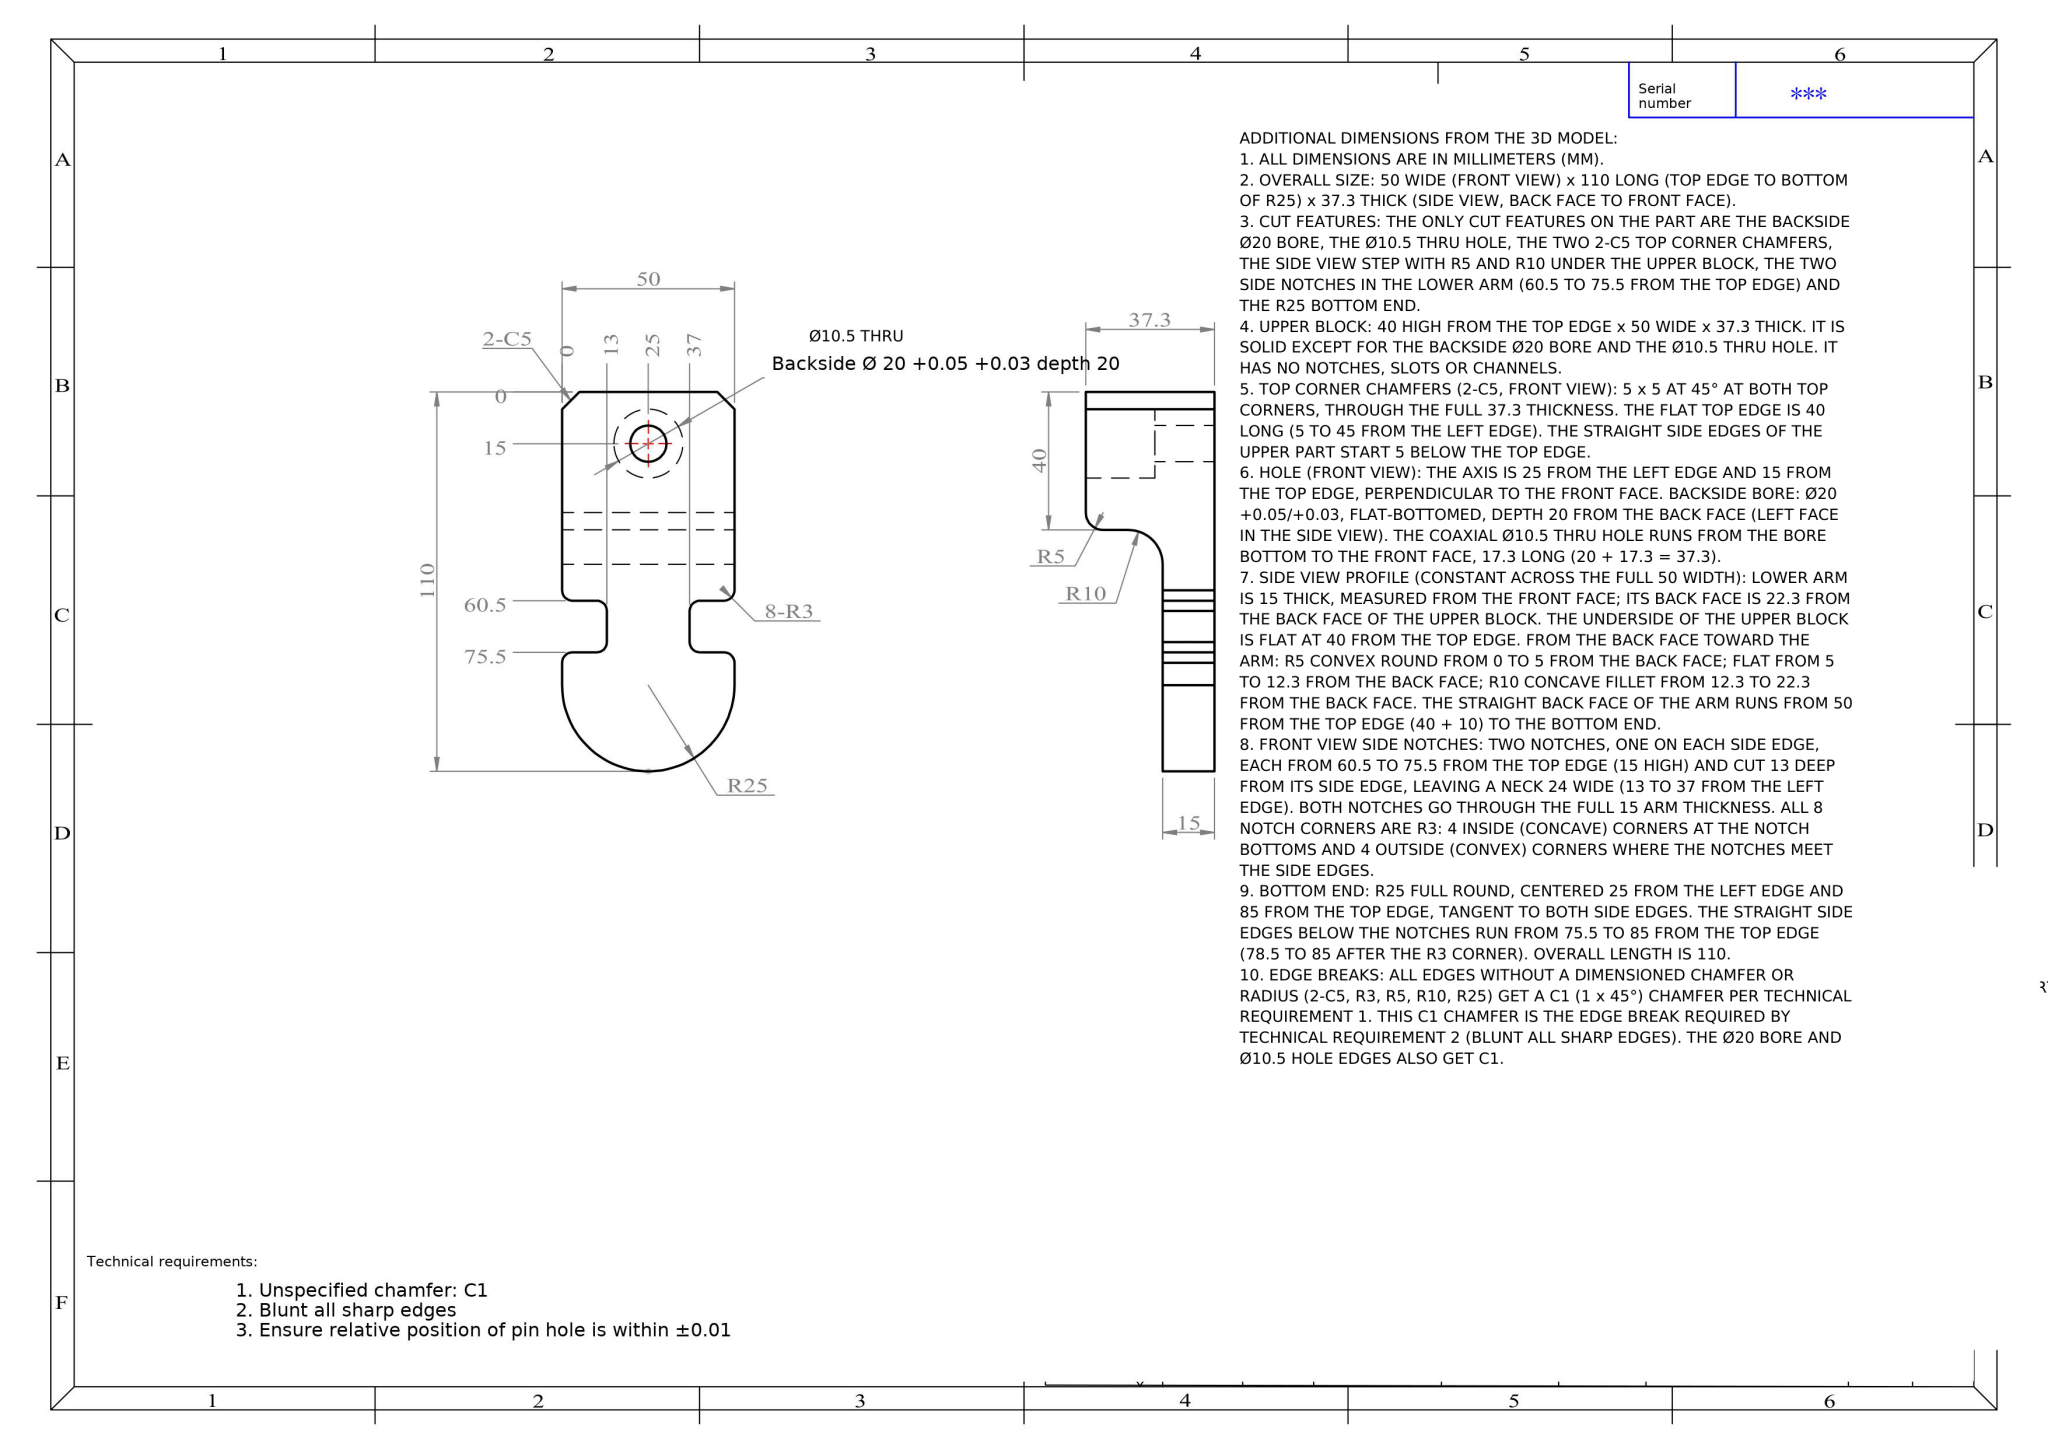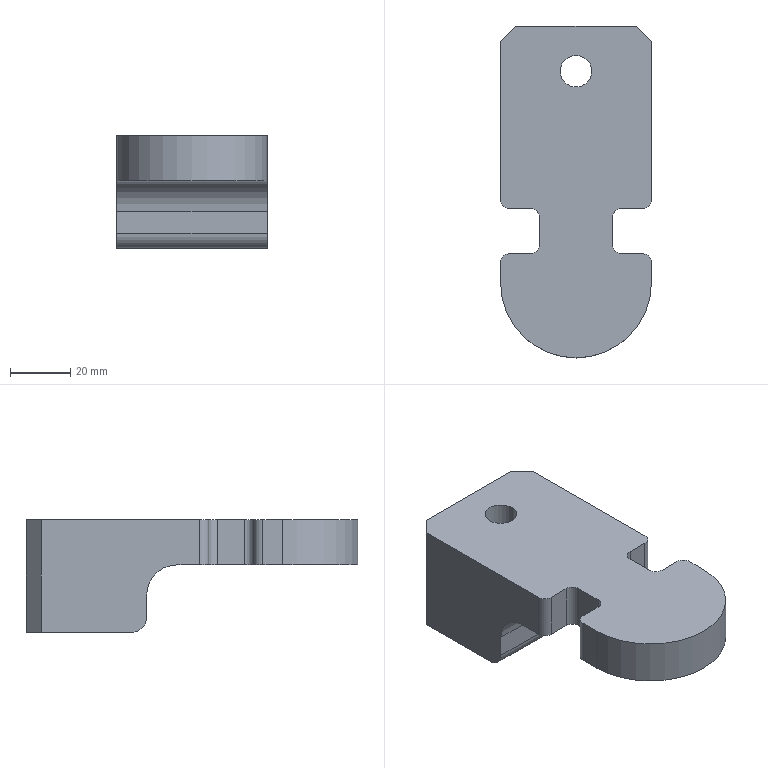Part | NX | mm | 1 solid | 33 faces | box 50 x 110 x 37.3 mm | volume 109317 mm3 | plane 18 | cylinder 15 | commonest cylinder face diameters 6 x8 20 x3 10.5 x2 10 x1 50 x1